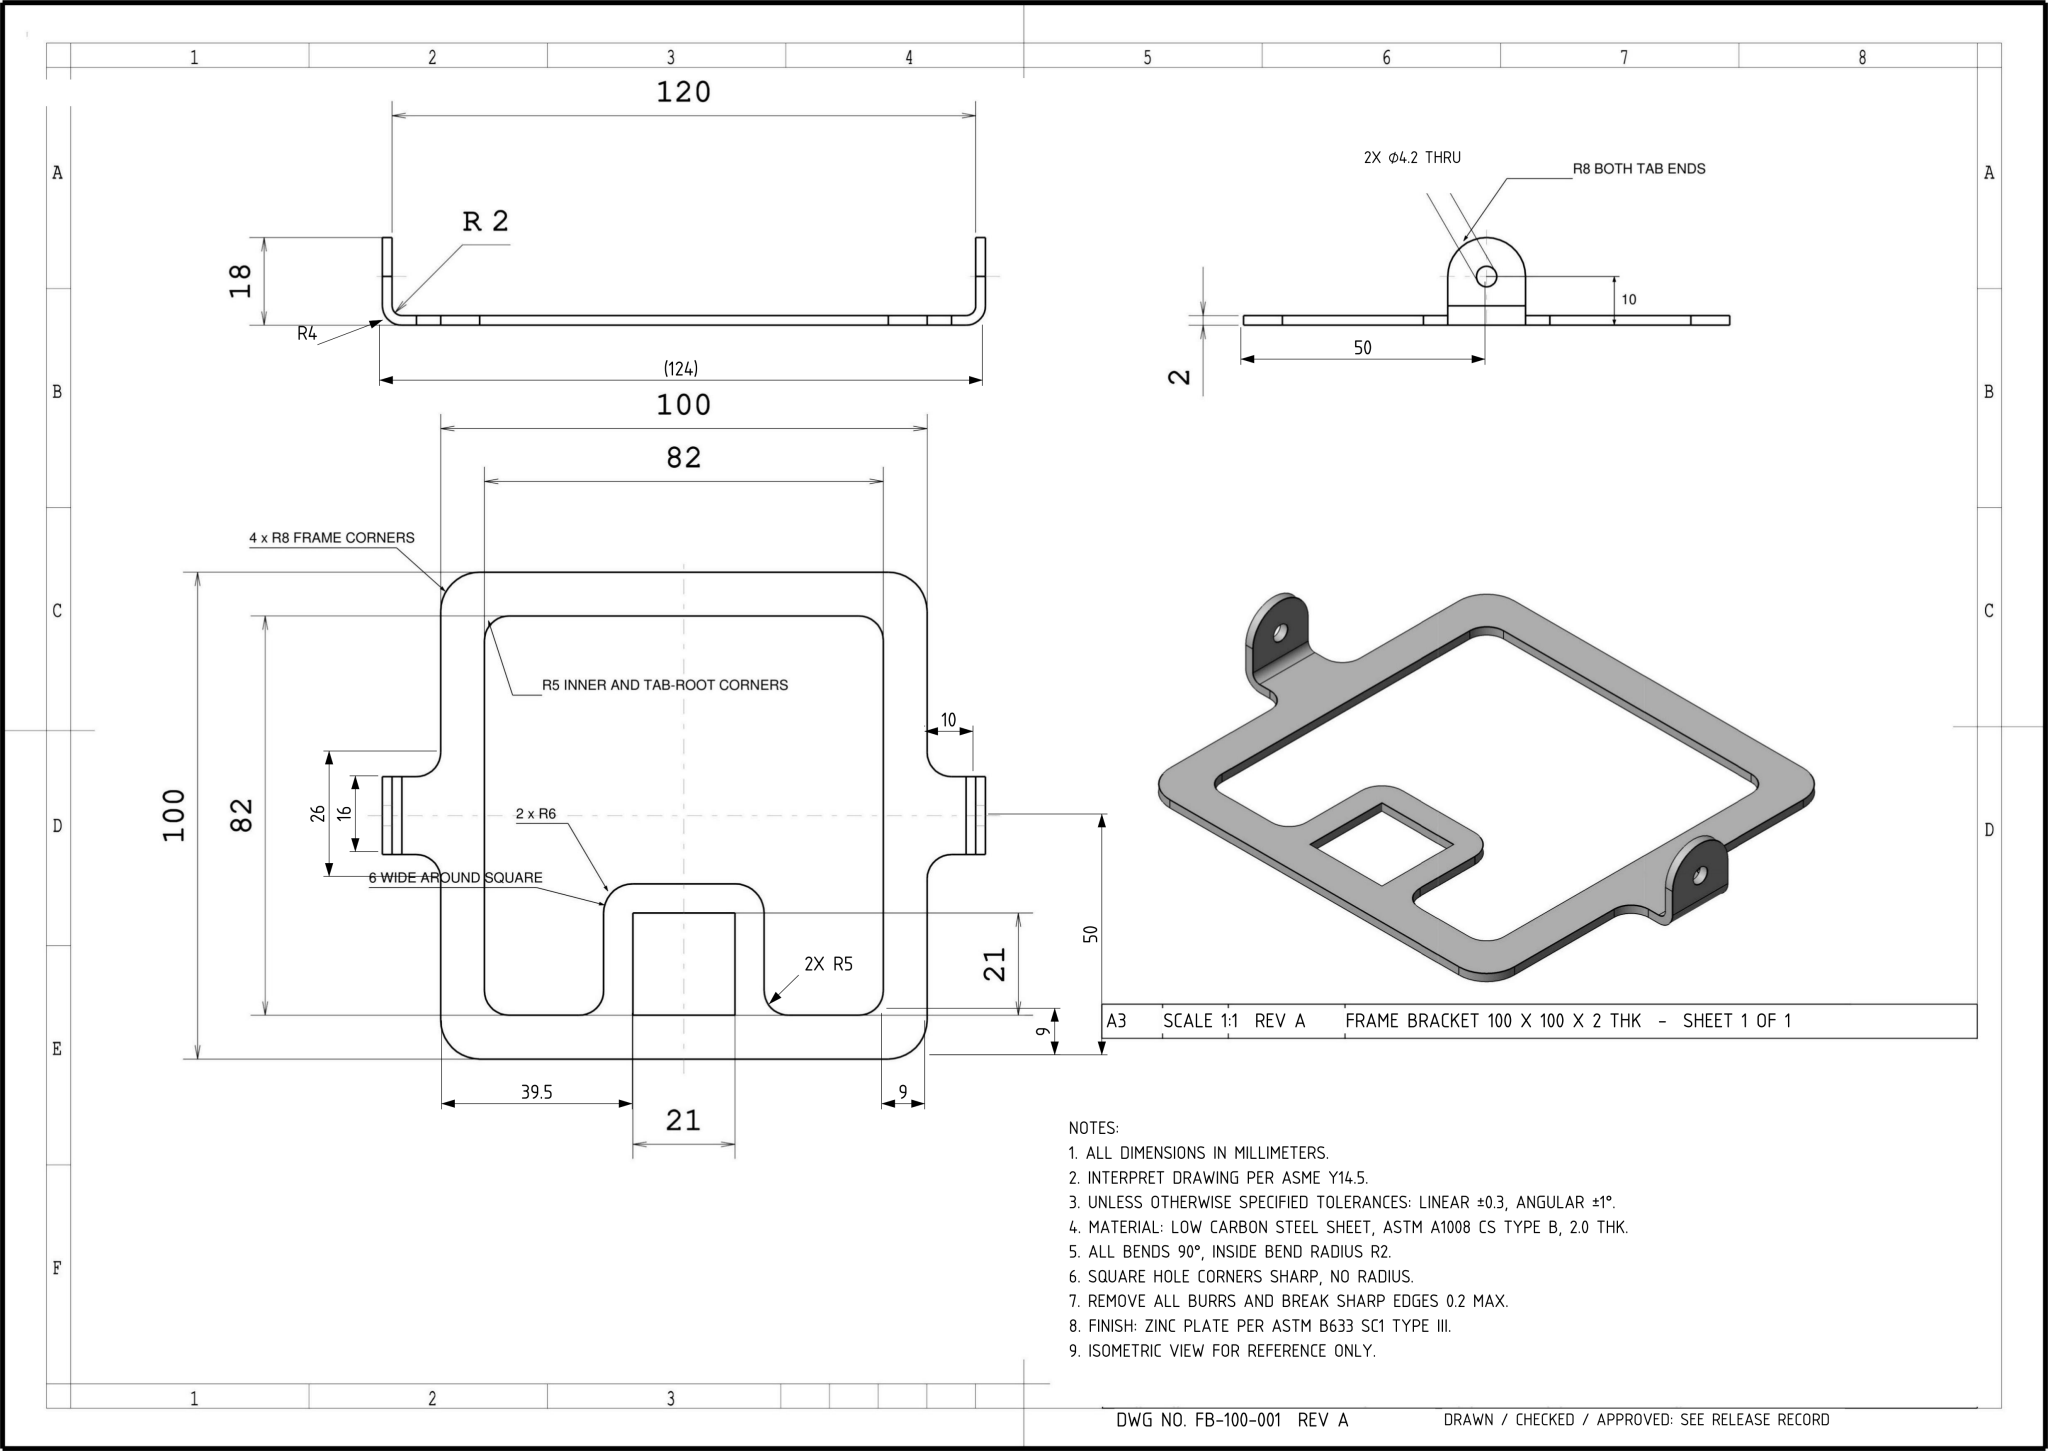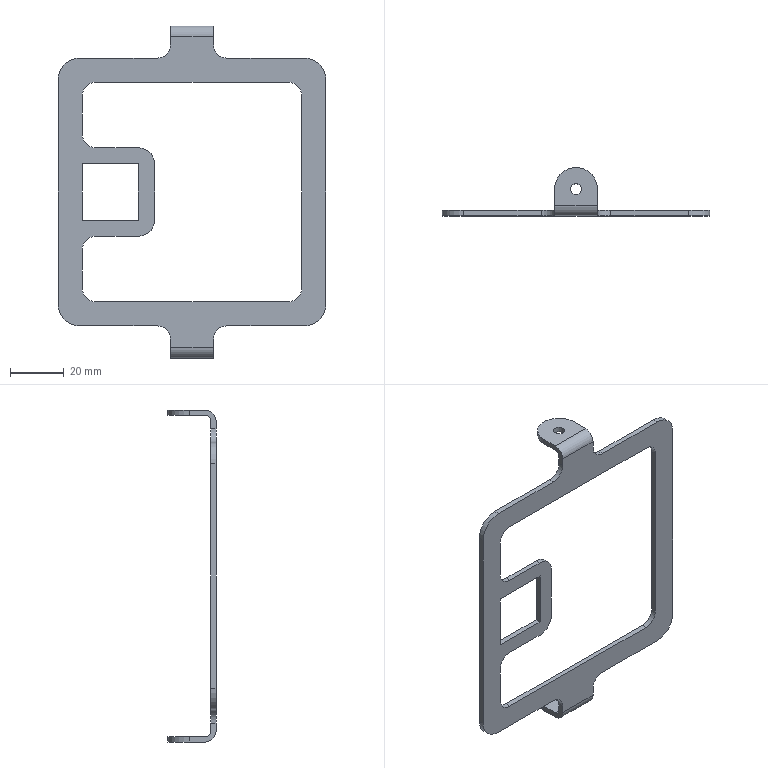Part | NX | mm | 1 solid | 52 faces | box 100 x 18 x 124 mm | volume 8963 mm3 | plane 28 | cylinder 24 | commonest cylinder face diameters 10 x10 16 x6 8 x2 4 x2 4.2 x2 12 x2